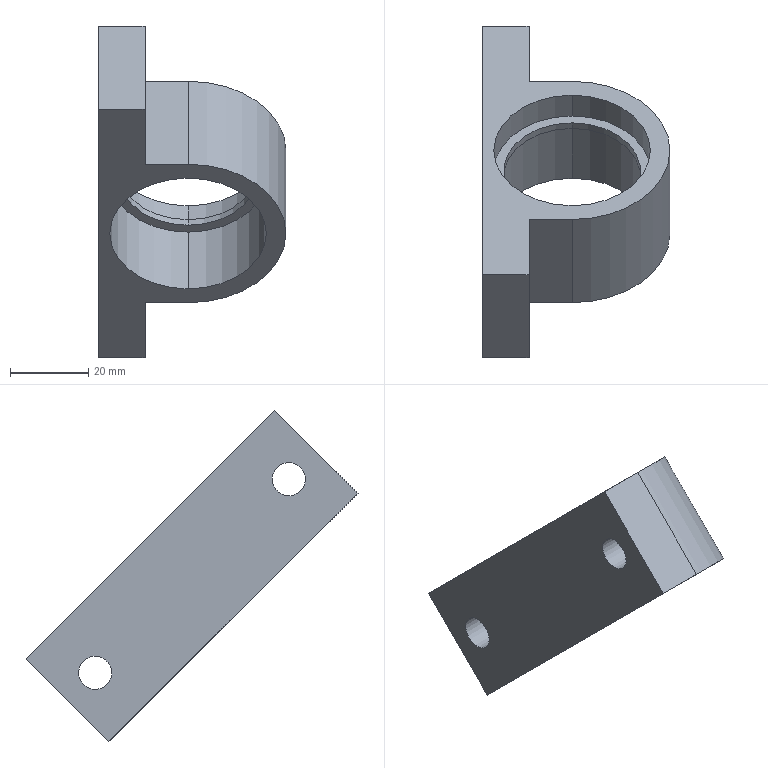Component | SolidWorks | AssemblyDriveAxis-1_BearingHousing6203-1 | 1 solid | 22 faces | box 48 x 84.85 x 84.85 mm | volume 39880 mm3 | cylinder 11 | plane 11 | commonest cylinder face diameters 40 x4 8.5 x4 35 x2 50 x1
build123d program:
from build123d import *

# Parameters (mm, degrees)
BOSS_EXTRUDE1_DEPTH            = 15
F_8_5_8_5_DIAMETER_HOLE1_D     = 8.5
F_8_5_8_5_DIAMETER_HOLE1_DEPTH = 52
F_8_5_8_5_DIAMETER_HOLE1_TIP   = 2.554
SKETCH6_R                      = 20
CUT_EXTRUDE1_DEPTH             = 7.5


with BuildPart() as part:
    # Sketch1 → Boss-Extrude1 (new, symmetric)
    with BuildSketch(Plane.XY):
        with BuildLine():
            Line((25, 17), (25, 6))
            Line((25, 6), (45, 6))
            Line((45, 6), (45, -6))
            Line((45, -6), (-45, -6))
            Line((-45, -6), (-45, 6))
            Line((-45, 6), (-25, 6))
            Line((-25, 6), (-25, 17))
            ThreePointArc((-25, 17), (0, 42), (25, 17))
        make_face()
    extrude(amount=BOSS_EXTRUDE1_DEPTH, both=True)

    # Sketch2 → Cut-Revolve1 (revolve, cut)
    with BuildSketch(Plane(origin=(0, 0, 0), x_dir=(0, 0, -1), z_dir=(1, 0, 0)), mode=Mode.PRIVATE) as cut_revolve1_sk:
        Polygon((15, 37), (8, 37), (6.5, 37), (-5.5, 37), (-5.5, 34.5), (-7.5, 34.5), (-7.5, 17), (15, 17), align=None)
    revolve(cut_revolve1_sk.sketch.rotate(Axis((0, 17, -34.227), (0, 0, 1)), 90), axis=Axis((0, 17, -34.227), (0, 0, 1)), mode=Mode.SUBTRACT)

    # 8.5 _8.5_ Diameter Hole1
    with Locations(Plane(origin=(0, 6, 0), x_dir=(1, 0, 0), z_dir=(0, 1, 0))):
        with Locations((35, 0), (-35, 0)):
            Hole(F_8_5_8_5_DIAMETER_HOLE1_D / 2, depth=F_8_5_8_5_DIAMETER_HOLE1_DEPTH)
            with Locations((0, 0, -(F_8_5_8_5_DIAMETER_HOLE1_DEPTH + F_8_5_8_5_DIAMETER_HOLE1_TIP / 2))):  # 118° drill point
                Cone(0, F_8_5_8_5_DIAMETER_HOLE1_D / 2, F_8_5_8_5_DIAMETER_HOLE1_TIP, mode=Mode.SUBTRACT)

    # Sketch6 → Cut-Extrude1 (cut)
    with BuildSketch(Plane.XY.offset(15)):
        with Locations(Location((0, 17, 0), (0, 0, 180))):
            Circle(SKETCH6_R)
    extrude(amount=-CUT_EXTRUDE1_DEPTH, mode=Mode.SUBTRACT)


solid = part.part

# Placed as in the assembly
solid = solid.moved(Location((-119, 778.165, 411.073), (-45, 0, -90)))
STEP:
#1=COLOUR_RGB('',0.7922,0.8196,0.9333);
#2=FILL_AREA_STYLE_COLOUR('',#1);
#3=FILL_AREA_STYLE('',(#2));
#4=SURFACE_STYLE_FILL_AREA(#3);
#5=SURFACE_SIDE_STYLE('',(#4));
#6=SURFACE_STYLE_USAGE(.BOTH.,#5);
#7=PRESENTATION_STYLE_ASSIGNMENT((#6));
#8=CARTESIAN_POINT('',(-4.016,31.402,15.836));
#9=VERTEX_POINT('',#8);
#10=CARTESIAN_POINT('',(-4.016,30.288,16.95));
#11=VERTEX_POINT('',#10);
#12=CARTESIAN_POINT('',(-4.016,30.845,16.393));
#13=DIRECTION('',(0.,0.7071,0.7071));
#14=DIRECTION('',(0.,-0.7071,0.7071));
#15=AXIS2_PLACEMENT_3D('',#12,#13,#14);
#16=CIRCLE('',#15,0.7874);
#17=EDGE_CURVE('',#9,#11,#16,.T.);
#18=ORIENTED_EDGE('',*,*,#17,.F.);
#19=CARTESIAN_POINT('',(-4.016,31.611,16.045));
#20=VERTEX_POINT('',#19);
#21=CARTESIAN_POINT('',(-4.016,31.402,15.836));
#22=DIRECTION('',(0.,0.7071,0.7071));
#23=VECTOR('',#22,39.37);
#24=LINE('',#21,#23);
#25=EDGE_CURVE('',#9,#20,#24,.T.);
#26=ORIENTED_EDGE('',*,*,#25,.T.);
#27=CARTESIAN_POINT('',(-4.016,30.497,17.158));
#28=VERTEX_POINT('',#27);
#29=CARTESIAN_POINT('',(-4.016,31.054,16.602));
#30=DIRECTION('',(0.,0.7071,0.7071));
#31=DIRECTION('',(0.,-0.7071,0.7071));
#32=AXIS2_PLACEMENT_3D('',#29,#30,#31);
#33=CIRCLE('',#32,0.7874);
#34=EDGE_CURVE('',#20,#28,#33,.T.);
#35=ORIENTED_EDGE('',*,*,#34,.T.);
#36=CARTESIAN_POINT('',(-4.016,30.288,16.95));
#37=DIRECTION('',(0.,0.7071,0.7071));
#38=VECTOR('',#37,39.37);
#39=LINE('',#36,#38);
#40=EDGE_CURVE('',#11,#28,#39,.T.);
#41=ORIENTED_EDGE('',*,*,#40,.F.);
#42=EDGE_LOOP('',(#18,#26,#35,#41));
#43=FACE_OUTER_BOUND('',#42,.T.);
#44=CARTESIAN_POINT('',(-4.016,30.845,16.393));
#45=DIRECTION('',(0.,0.7071,0.7071));
#46=DIRECTION('',(0.,-0.7071,0.7071));
#47=AXIS2_PLACEMENT_3D('',#44,#45,#46);
#48=CYLINDRICAL_SURFACE('',#47,0.7874);
#49=ADVANCED_FACE('',(#43),#48,.F.);
#50=CARTESIAN_POINT('',(-4.921,29.544,17.04));
#51=VERTEX_POINT('',#50);
#52=CARTESIAN_POINT('',(-4.921,29.78,17.277));
#53=VERTEX_POINT('',#52);
#54=CARTESIAN_POINT('',(-4.921,29.662,17.158));
#55=DIRECTION('',(1.,-0.,0.));
#56=DIRECTION('',(0.,0.7071,0.7071));
#57=AXIS2_PLACEMENT_3D('',#54,#55,#56);
#58=CIRCLE('',#57,0.1673);
#59=EDGE_CURVE('',#51,#53,#58,.T.);
#60=ORIENTED_EDGE('',*,*,#59,.F.);
#61=CARTESIAN_POINT('',(-4.449,29.544,17.04));
#62=VERTEX_POINT('',#61);
#63=CARTESIAN_POINT('',(-4.449,29.544,17.04));
#64=DIRECTION('',(1.,-0.,0.));
#65=VECTOR('',#64,39.37);
#66=LINE('',#63,#65);
#67=EDGE_CURVE('',#51,#62,#66,.T.);
#68=ORIENTED_EDGE('',*,*,#67,.T.);
#69=CARTESIAN_POINT('',(-4.449,29.78,17.277));
#70=VERTEX_POINT('',#69);
#71=CARTESIAN_POINT('',(-4.449,29.662,17.158));
#72=DIRECTION('',(1.,-0.,0.));
#73=DIRECTION('',(0.,0.7071,0.7071));
#74=AXIS2_PLACEMENT_3D('',#71,#72,#73);
#75=CIRCLE('',#74,0.1673);
#76=EDGE_CURVE('',#62,#70,#75,.T.);
#77=ORIENTED_EDGE('',*,*,#76,.T.);
#78=CARTESIAN_POINT('',(-4.449,29.78,17.277));
#79=DIRECTION('',(1.,-0.,0.));
#80=VECTOR('',#79,39.37);
#81=LINE('',#78,#80);
#82=EDGE_CURVE('',#53,#70,#81,.T.);
#83=ORIENTED_EDGE('',*,*,#82,.F.);
#84=EDGE_LOOP('',(#60,#68,#77,#83));
#85=FACE_OUTER_BOUND('',#84,.T.);
#86=CARTESIAN_POINT('',(-4.449,29.662,17.158));
#87=DIRECTION('',(1.,-0.,0.));
#88=DIRECTION('',(0.,0.7071,0.7071));
#89=AXIS2_PLACEMENT_3D('',#86,#87,#88);
#90=CYLINDRICAL_SURFACE('',#89,0.1673);
#91=ADVANCED_FACE('',(#85),#90,.F.);
#92=CARTESIAN_POINT('',(-4.921,31.492,15.091));
#93=VERTEX_POINT('',#92);
#94=CARTESIAN_POINT('',(-4.921,31.729,15.328));
#95=VERTEX_POINT('',#94);
#96=CARTESIAN_POINT('',(-4.921,31.611,15.21));
#97=DIRECTION('',(1.,-0.,0.));
#98=DIRECTION('',(0.,0.7071,0.7071));
#99=AXIS2_PLACEMENT_3D('',#96,#97,#98);
#100=CIRCLE('',#99,0.1673);
#101=EDGE_CURVE('',#93,#95,#100,.T.);
#102=ORIENTED_EDGE('',*,*,#101,.F.);
#103=CARTESIAN_POINT('',(-4.449,31.492,15.091));
#104=VERTEX_POINT('',#103);
#105=CARTESIAN_POINT('',(-4.449,31.492,15.091));
#106=DIRECTION('',(1.,-0.,0.));
#107=VECTOR('',#106,39.37);
#108=LINE('',#105,#107);
#109=EDGE_CURVE('',#93,#104,#108,.T.);
#110=ORIENTED_EDGE('',*,*,#109,.T.);
#111=CARTESIAN_POINT('',(-4.449,31.729,15.328));
#112=VERTEX_POINT('',#111);
#113=CARTESIAN_POINT('',(-4.449,31.611,15.21));
#114=DIRECTION('',(1.,-0.,0.));
#115=DIRECTION('',(0.,0.7071,0.7071));
#116=AXIS2_PLACEMENT_3D('',#113,#114,#115);
#117=CIRCLE('',#116,0.1673);
#118=EDGE_CURVE('',#104,#112,#117,.T.);
#119=ORIENTED_EDGE('',*,*,#118,.T.);
#120=CARTESIAN_POINT('',(-4.449,31.729,15.328));
#121=DIRECTION('',(1.,-0.,0.));
#122=VECTOR('',#121,39.37);
#123=LINE('',#120,#122);
#124=EDGE_CURVE('',#95,#112,#123,.T.);
#125=ORIENTED_EDGE('',*,*,#124,.F.);
#126=EDGE_LOOP('',(#102,#110,#119,#125));
#127=FACE_OUTER_BOUND('',#126,.T.);
#128=CARTESIAN_POINT('',(-4.449,31.611,15.21));
#129=DIRECTION('',(1.,-0.,0.));
#130=DIRECTION('',(0.,0.7071,0.7071));
#131=AXIS2_PLACEMENT_3D('',#128,#129,#130);
#132=CYLINDRICAL_SURFACE('',#131,0.1673);
#133=ADVANCED_FACE('',(#127),#132,.F.);
#134=CARTESIAN_POINT('',(-4.016,30.358,16.88));
#135=VERTEX_POINT('',#134);
#136=CARTESIAN_POINT('',(-4.016,31.332,15.906));
#137=VERTEX_POINT('',#136);
#138=CARTESIAN_POINT('',(-4.016,30.845,16.393));
#139=DIRECTION('',(0.,-0.7071,-0.7071));
#140=DIRECTION('',(0.,0.7071,-0.7071));
#141=AXIS2_PLACEMENT_3D('',#138,#139,#140);
#142=CIRCLE('',#141,0.689);
#143=EDGE_CURVE('',#135,#137,#142,.T.);
#144=ORIENTED_EDGE('',*,*,#143,.F.);
#145=CARTESIAN_POINT('',(-4.016,30.302,16.824));
#146=VERTEX_POINT('',#145);
#147=CARTESIAN_POINT('',(-4.016,29.196,15.718));
#148=DIRECTION('',(0.,-0.7071,-0.7071));
#149=VECTOR('',#148,39.37);
#150=LINE('',#147,#149);
#151=EDGE_CURVE('',#135,#146,#150,.T.);
#152=ORIENTED_EDGE('',*,*,#151,.T.);
#153=CARTESIAN_POINT('',(-4.016,31.277,15.85));
#154=VERTEX_POINT('',#153);
#155=CARTESIAN_POINT('',(-4.016,30.79,16.337));
#156=DIRECTION('',(0.,-0.7071,-0.7071));
#157=DIRECTION('',(0.,0.7071,-0.7071));
#158=AXIS2_PLACEMENT_3D('',#155,#156,#157);
#159=CIRCLE('',#158,0.689);
#160=EDGE_CURVE('',#146,#154,#159,.T.);
#161=ORIENTED_EDGE('',*,*,#160,.T.);
#162=CARTESIAN_POINT('',(-4.016,30.171,14.744));
#163=DIRECTION('',(0.,-0.7071,-0.7071));
#164=VECTOR('',#163,39.37);
#165=LINE('',#162,#164);
#166=EDGE_CURVE('',#137,#154,#165,.T.);
#167=ORIENTED_EDGE('',*,*,#166,.F.);
#168=EDGE_LOOP('',(#144,#152,#161,#167));
#169=FACE_OUTER_BOUND('',#168,.T.);
#170=CARTESIAN_POINT('',(-4.016,29.684,15.231));
#171=DIRECTION('',(0.,-0.7071,-0.7071));
#172=DIRECTION('',(0.,0.7071,-0.7071));
#173=AXIS2_PLACEMENT_3D('',#170,#171,#172);
#174=CYLINDRICAL_SURFACE('',#173,0.689);
#175=ADVANCED_FACE('',(#169),#174,.F.);
#176=CARTESIAN_POINT('',(-4.016,30.233,16.894));
#177=VERTEX_POINT('',#176);
#178=CARTESIAN_POINT('',(-4.016,31.346,15.78));
#179=VERTEX_POINT('',#178);
#180=CARTESIAN_POINT('',(-4.016,30.79,16.337));
#181=DIRECTION('',(0.,-0.7071,-0.7071));
#182=DIRECTION('',(0.,0.7071,-0.7071));
#183=AXIS2_PLACEMENT_3D('',#180,#181,#182);
#184=CIRCLE('',#183,0.7874);
#185=EDGE_CURVE('',#177,#179,#184,.T.);
#186=ORIENTED_EDGE('',*,*,#185,.F.);
#187=CARTESIAN_POINT('',(-4.016,29.662,16.323));
#188=VERTEX_POINT('',#187);
#189=CARTESIAN_POINT('',(-4.016,29.127,15.788));
#190=DIRECTION('',(0.,-0.7071,-0.7071));
#191=VECTOR('',#190,39.37);
#192=LINE('',#189,#191);
#193=EDGE_CURVE('',#177,#188,#192,.T.);
#194=ORIENTED_EDGE('',*,*,#193,.T.);
#195=CARTESIAN_POINT('',(-4.016,30.776,15.21));
#196=VERTEX_POINT('',#195);
#197=CARTESIAN_POINT('',(-4.016,30.219,15.766));
#198=DIRECTION('',(0.,-0.7071,-0.7071));
#199=DIRECTION('',(0.,0.7071,-0.7071));
#200=AXIS2_PLACEMENT_3D('',#197,#198,#199);
#201=CIRCLE('',#200,0.7874);
#202=EDGE_CURVE('',#188,#196,#201,.T.);
#203=ORIENTED_EDGE('',*,*,#202,.T.);
#204=CARTESIAN_POINT('',(-4.016,30.24,14.674));
#205=DIRECTION('',(0.,-0.7071,-0.7071));
#206=VECTOR('',#205,39.37);
#207=LINE('',#204,#206);
#208=EDGE_CURVE('',#179,#196,#207,.T.);
#209=ORIENTED_EDGE('',*,*,#208,.F.);
#210=EDGE_LOOP('',(#186,#194,#203,#209));
#211=FACE_OUTER_BOUND('',#210,.T.);
#212=CARTESIAN_POINT('',(-4.016,29.684,15.231));
#213=DIRECTION('',(0.,-0.7071,-0.7071));
#214=DIRECTION('',(0.,0.7071,-0.7071));
#215=AXIS2_PLACEMENT_3D('',#212,#213,#214);
#216=CYLINDRICAL_SURFACE('',#215,0.7874);
#217=ADVANCED_FACE('',(#211),#216,.F.);
#218=CARTESIAN_POINT('',(-4.921,28.966,17.019));
#219=VERTEX_POINT('',#218);
#220=CARTESIAN_POINT('',(-4.449,28.966,17.019));
#221=VERTEX_POINT('',#220);
#222=CARTESIAN_POINT('',(-4.449,28.966,17.019));
#223=DIRECTION('',(1.,-0.,0.));
#224=VECTOR('',#223,39.37);
#225=LINE('',#222,#224);
#226=EDGE_CURVE('',#219,#221,#225,.T.);
#227=ORIENTED_EDGE('',*,*,#226,.T.);
#228=CARTESIAN_POINT('',(-4.449,29.801,17.854));
#229=VERTEX_POINT('',#228);
#230=CARTESIAN_POINT('',(-4.449,29.801,17.854));
#231=DIRECTION('',(0.,-0.7071,-0.7071));
#232=VECTOR('',#231,39.37);
#233=LINE('',#230,#232);
#234=EDGE_CURVE('',#229,#221,#233,.T.);
#235=ORIENTED_EDGE('',*,*,#234,.F.);
#236=CARTESIAN_POINT('',(-4.921,29.801,17.854));
#237=VERTEX_POINT('',#236);
#238=CARTESIAN_POINT('',(-4.449,29.801,17.854));
#239=DIRECTION('',(1.,-0.,0.));
#240=VECTOR('',#239,39.37);
#241=LINE('',#238,#240);
#242=EDGE_CURVE('',#237,#229,#241,.T.);
#243=ORIENTED_EDGE('',*,*,#242,.F.);
#244=CARTESIAN_POINT('',(-4.921,29.801,17.854));
#245=DIRECTION('',(0.,-0.7071,-0.7071));
#246=VECTOR('',#245,39.37);
#247=LINE('',#244,#246);
#248=EDGE_CURVE('',#237,#219,#247,.T.);
#249=ORIENTED_EDGE('',*,*,#248,.T.);
#250=EDGE_LOOP('',(#227,#235,#243,#249));
#251=FACE_OUTER_BOUND('',#250,.T.);
#252=CARTESIAN_POINT('',(-4.449,29.801,17.854));
#253=DIRECTION('',(0.,0.7071,-0.7071));
#254=DIRECTION('',(0.,0.7071,0.7071));
#255=AXIS2_PLACEMENT_3D('',#252,#253,#254);
#256=PLANE('',#255);
#257=ADVANCED_FACE('',(#251),#256,.F.);
#258=CARTESIAN_POINT('',(-4.449,29.662,17.158));
#259=DIRECTION('',(1.,-0.,0.));
#260=DIRECTION('',(0.,0.7071,0.7071));
#261=AXIS2_PLACEMENT_3D('',#258,#259,#260);
#262=CIRCLE('',#261,0.1673);
#263=EDGE_CURVE('',#70,#62,#262,.T.);
#264=ORIENTED_EDGE('',*,*,#263,.F.);
#265=ORIENTED_EDGE('',*,*,#76,.F.);
#266=EDGE_LOOP('',(#264,#265));
#267=FACE_BOUND('',#266,.T.);
#268=CARTESIAN_POINT('',(-4.449,29.523,16.462));
#269=VERTEX_POINT('',#268);
#270=CARTESIAN_POINT('',(-4.449,29.523,16.462));
#271=DIRECTION('',(0.,0.7071,-0.7071));
#272=VECTOR('',#271,39.37);
#273=LINE('',#270,#272);
#274=EDGE_CURVE('',#221,#269,#273,.T.);
#275=ORIENTED_EDGE('',*,*,#274,.T.);
#276=CARTESIAN_POINT('',(-4.449,30.358,17.298));
#277=VERTEX_POINT('',#276);
#278=CARTESIAN_POINT('',(-4.449,30.358,17.298));
#279=DIRECTION('',(0.,-0.7071,-0.7071));
#280=VECTOR('',#279,39.37);
#281=LINE('',#278,#280);
#282=EDGE_CURVE('',#277,#269,#281,.T.);
#283=ORIENTED_EDGE('',*,*,#282,.F.);
#284=CARTESIAN_POINT('',(-4.449,30.358,17.298));
#285=DIRECTION('',(0.,0.7071,-0.7071));
#286=VECTOR('',#285,39.37);
#287=LINE('',#284,#286);
#288=EDGE_CURVE('',#229,#277,#287,.T.);
#289=ORIENTED_EDGE('',*,*,#288,.F.);
#290=ORIENTED_EDGE('',*,*,#234,.T.);
#291=EDGE_LOOP('',(#275,#283,#289,#290));
#292=FACE_OUTER_BOUND('',#291,.T.);
#293=CARTESIAN_POINT('',(-4.449,30.358,17.298));
#294=DIRECTION('',(-1.,0.,-0.));
#295=DIRECTION('',(-0.,-0.7071,0.7071));
#296=AXIS2_PLACEMENT_3D('',#293,#294,#295);
#297=PLANE('',#296);
#298=ADVANCED_FACE('',(#267,#292),#297,.F.);
#299=CARTESIAN_POINT('',(-4.016,29.523,16.462));
#300=VERTEX_POINT('',#299);
#301=CARTESIAN_POINT('',(-4.016,29.523,16.462));
#302=DIRECTION('',(1.,-0.,0.));
#303=VECTOR('',#302,39.37);
#304=LINE('',#301,#303);
#305=EDGE_CURVE('',#269,#300,#304,.T.);
#306=ORIENTED_EDGE('',*,*,#305,.T.);
#307=CARTESIAN_POINT('',(-4.016,30.358,17.298));
#308=VERTEX_POINT('',#307);
#309=CARTESIAN_POINT('',(-4.016,30.358,17.298));
#310=DIRECTION('',(0.,-0.7071,-0.7071));
#311=VECTOR('',#310,39.37);
#312=LINE('',#309,#311);
#313=EDGE_CURVE('',#308,#300,#312,.T.);
#314=ORIENTED_EDGE('',*,*,#313,.F.);
#315=CARTESIAN_POINT('',(-4.016,30.358,17.298));
#316=DIRECTION('',(1.,-0.,0.));
#317=VECTOR('',#316,39.37);
#318=LINE('',#315,#317);
#319=EDGE_CURVE('',#277,#308,#318,.T.);
#320=ORIENTED_EDGE('',*,*,#319,.F.);
#321=ORIENTED_EDGE('',*,*,#282,.T.);
#322=EDGE_LOOP('',(#306,#314,#320,#321));
#323=FACE_OUTER_BOUND('',#322,.T.);
#324=CARTESIAN_POINT('',(-4.016,30.358,17.298));
#325=DIRECTION('',(0.,0.7071,-0.7071));
#326=DIRECTION('',(-1.,0.,-0.));
#327=AXIS2_PLACEMENT_3D('',#324,#325,#326);
#328=PLANE('',#327);
#329=ADVANCED_FACE('',(#323),#328,.F.);
#330=CARTESIAN_POINT('',(-4.016,30.915,15.07));
#331=VERTEX_POINT('',#330);
#332=CARTESIAN_POINT('',(-4.016,30.219,15.766));
#333=DIRECTION('',(0.,0.7071,0.7071));
#334=DIRECTION('',(0.,-0.7071,0.7071));
#335=AXIS2_PLACEMENT_3D('',#332,#333,#334);
#336=CIRCLE('',#335,0.9843);
#337=EDGE_CURVE('',#300,#331,#336,.T.);
#338=ORIENTED_EDGE('',*,*,#337,.T.);
#339=CARTESIAN_POINT('',(-4.016,31.75,15.906));
#340=VERTEX_POINT('',#339);
#341=CARTESIAN_POINT('',(-4.016,31.75,15.906));
#342=DIRECTION('',(0.,-0.7071,-0.7071));
#343=VECTOR('',#342,39.37);
#344=LINE('',#341,#343);
#345=EDGE_CURVE('',#340,#331,#344,.T.);
#346=ORIENTED_EDGE('',*,*,#345,.F.);
#347=CARTESIAN_POINT('',(-4.016,31.054,16.602));
#348=DIRECTION('',(0.,0.7071,0.7071));
#349=DIRECTION('',(0.,-0.7071,0.7071));
#350=AXIS2_PLACEMENT_3D('',#347,#348,#349);
#351=CIRCLE('',#350,0.9843);
#352=EDGE_CURVE('',#308,#340,#351,.T.);
#353=ORIENTED_EDGE('',*,*,#352,.F.);
#354=ORIENTED_EDGE('',*,*,#313,.T.);
#355=EDGE_LOOP('',(#338,#346,#353,#354));
#356=FACE_OUTER_BOUND('',#355,.T.);
#357=CARTESIAN_POINT('',(-4.016,31.054,16.602));
#358=DIRECTION('',(0.,-0.7071,-0.7071));
#359=DIRECTION('',(0.,0.7071,-0.7071));
#360=AXIS2_PLACEMENT_3D('',#357,#358,#359);
#361=CYLINDRICAL_SURFACE('',#360,0.9843);
#362=ADVANCED_FACE('',(#356),#361,.T.);
#363=CARTESIAN_POINT('',(-4.449,30.915,15.07));
#364=VERTEX_POINT('',#363);
#365=CARTESIAN_POINT('',(-4.016,30.915,15.07));
#366=DIRECTION('',(-1.,-0.,0.));
#367=VECTOR('',#366,39.37);
#368=LINE('',#365,#367);
#369=EDGE_CURVE('',#331,#364,#368,.T.);
#370=ORIENTED_EDGE('',*,*,#369,.T.);
#371=CARTESIAN_POINT('',(-4.449,31.75,15.906));
#372=VERTEX_POINT('',#371);
#373=CARTESIAN_POINT('',(-4.449,31.75,15.906));
#374=DIRECTION('',(0.,-0.7071,-0.7071));
#375=VECTOR('',#374,39.37);
#376=LINE('',#373,#375);
#377=EDGE_CURVE('',#372,#364,#376,.T.);
#378=ORIENTED_EDGE('',*,*,#377,.F.);
#379=CARTESIAN_POINT('',(-4.016,31.75,15.906));
#380=DIRECTION('',(-1.,-0.,0.));
#381=VECTOR('',#380,39.37);
#382=LINE('',#379,#381);
#383=EDGE_CURVE('',#340,#372,#382,.T.);
#384=ORIENTED_EDGE('',*,*,#383,.F.);
#385=ORIENTED_EDGE('',*,*,#345,.T.);
#386=EDGE_LOOP('',(#370,#378,#384,#385));
#387=FACE_OUTER_BOUND('',#386,.T.);
#388=CARTESIAN_POINT('',(-4.016,31.75,15.906));
#389=DIRECTION('',(0.,-0.7071,0.7071));
#390=DIRECTION('',(1.,0.,-0.));
#391=AXIS2_PLACEMENT_3D('',#388,#389,#390);
#392=PLANE('',#391);
#393=ADVANCED_FACE('',(#387),#392,.F.);
#394=CARTESIAN_POINT('',(-4.449,31.611,15.21));
#395=DIRECTION('',(1.,-0.,0.));
#396=DIRECTION('',(0.,0.7071,0.7071));
#397=AXIS2_PLACEMENT_3D('',#394,#395,#396);
#398=CIRCLE('',#397,0.1673);
#399=EDGE_CURVE('',#112,#104,#398,.T.);
#400=ORIENTED_EDGE('',*,*,#399,.F.);
#401=ORIENTED_EDGE('',*,*,#118,.F.);
#402=EDGE_LOOP('',(#400,#401));
#403=FACE_BOUND('',#402,.T.);
#404=CARTESIAN_POINT('',(-4.449,31.472,14.514));
#405=VERTEX_POINT('',#404);
#406=CARTESIAN_POINT('',(-4.449,31.472,14.514));
#407=DIRECTION('',(0.,0.7071,-0.7071));
#408=VECTOR('',#407,39.37);
#409=LINE('',#406,#408);
#410=EDGE_CURVE('',#364,#405,#409,.T.);
#411=ORIENTED_EDGE('',*,*,#410,.T.);
#412=CARTESIAN_POINT('',(-4.449,32.307,15.349));
#413=VERTEX_POINT('',#412);
#414=CARTESIAN_POINT('',(-4.449,32.307,15.349));
#415=DIRECTION('',(0.,-0.7071,-0.7071));
#416=VECTOR('',#415,39.37);
#417=LINE('',#414,#416);
#418=EDGE_CURVE('',#413,#405,#417,.T.);
#419=ORIENTED_EDGE('',*,*,#418,.F.);
#420=CARTESIAN_POINT('',(-4.449,32.307,15.349));
#421=DIRECTION('',(0.,0.7071,-0.7071));
#422=VECTOR('',#421,39.37);
#423=LINE('',#420,#422);
#424=EDGE_CURVE('',#372,#413,#423,.T.);
#425=ORIENTED_EDGE('',*,*,#424,.F.);
#426=ORIENTED_EDGE('',*,*,#377,.T.);
#427=EDGE_LOOP('',(#411,#419,#425,#426));
#428=FACE_OUTER_BOUND('',#427,.T.);
#429=CARTESIAN_POINT('',(-4.449,32.307,15.349));
#430=DIRECTION('',(-1.,0.,-0.));
#431=DIRECTION('',(0.,-0.7071,-0.7071));
#432=AXIS2_PLACEMENT_3D('',#429,#430,#431);
#433=PLANE('',#432);
#434=ADVANCED_FACE('',(#403,#428),#433,.F.);
#435=CARTESIAN_POINT('',(-4.921,31.472,14.514));
#436=VERTEX_POINT('',#435);
#437=CARTESIAN_POINT('',(-4.449,31.472,14.514));
#438=DIRECTION('',(-1.,0.,-0.));
#439=VECTOR('',#438,39.37);
#440=LINE('',#437,#439);
#441=EDGE_CURVE('',#405,#436,#440,.T.);
#442=ORIENTED_EDGE('',*,*,#441,.T.);
#443=CARTESIAN_POINT('',(-4.921,32.307,15.349));
#444=VERTEX_POINT('',#443);
#445=CARTESIAN_POINT('',(-4.921,32.307,15.349));
#446=DIRECTION('',(0.,-0.7071,-0.7071));
#447=VECTOR('',#446,39.37);
#448=LINE('',#445,#447);
#449=EDGE_CURVE('',#444,#436,#448,.T.);
#450=ORIENTED_EDGE('',*,*,#449,.F.);
#451=CARTESIAN_POINT('',(-4.449,32.307,15.349));
#452=DIRECTION('',(-1.,0.,-0.));
#453=VECTOR('',#452,39.37);
#454=LINE('',#451,#453);
#455=EDGE_CURVE('',#413,#444,#454,.T.);
#456=ORIENTED_EDGE('',*,*,#455,.F.);
#457=ORIENTED_EDGE('',*,*,#418,.T.);
#458=EDGE_LOOP('',(#442,#450,#456,#457));
#459=FACE_OUTER_BOUND('',#458,.T.);
#460=CARTESIAN_POINT('',(-4.449,32.307,15.349));
#461=DIRECTION('',(-0.,-0.7071,0.7071));
#462=DIRECTION('',(0.,-0.7071,-0.7071));
#463=AXIS2_PLACEMENT_3D('',#460,#461,#462);
#464=PLANE('',#463);
#465=ADVANCED_FACE('',(#459),#464,.F.);
#466=CARTESIAN_POINT('',(-4.921,29.662,17.158));
#467=DIRECTION('',(1.,-0.,0.));
#468=DIRECTION('',(0.,0.7071,0.7071));
#469=AXIS2_PLACEMENT_3D('',#466,#467,#468);
#470=CIRCLE('',#469,0.1673);
#471=EDGE_CURVE('',#53,#51,#470,.T.);
#472=ORIENTED_EDGE('',*,*,#471,.T.);
#473=ORIENTED_EDGE('',*,*,#59,.T.);
#474=EDGE_LOOP('',(#472,#473));
#475=FACE_BOUND('',#474,.T.);
#476=CARTESIAN_POINT('',(-4.921,31.611,15.21));
#477=DIRECTION('',(1.,-0.,0.));
#478=DIRECTION('',(0.,0.7071,0.7071));
#479=AXIS2_PLACEMENT_3D('',#476,#477,#478);
#480=CIRCLE('',#479,0.1673);
#481=EDGE_CURVE('',#95,#93,#480,.T.);
#482=ORIENTED_EDGE('',*,*,#481,.T.);
#483=ORIENTED_EDGE('',*,*,#101,.T.);
#484=EDGE_LOOP('',(#482,#483));
#485=FACE_BOUND('',#484,.T.);
#486=CARTESIAN_POINT('',(-4.921,31.472,14.514));
#487=DIRECTION('',(-0.,-0.7071,0.7071));
#488=VECTOR('',#487,39.37);
#489=LINE('',#486,#488);
#490=EDGE_CURVE('',#436,#219,#489,.T.);
#491=ORIENTED_EDGE('',*,*,#490,.T.);
#492=ORIENTED_EDGE('',*,*,#248,.F.);
#493=CARTESIAN_POINT('',(-4.921,32.307,15.349));
#494=DIRECTION('',(-0.,-0.7071,0.7071));
#495=VECTOR('',#494,39.37);
#496=LINE('',#493,#495);
#497=EDGE_CURVE('',#444,#237,#496,.T.);
#498=ORIENTED_EDGE('',*,*,#497,.F.);
#499=ORIENTED_EDGE('',*,*,#449,.T.);
#500=EDGE_LOOP('',(#491,#492,#498,#499));
#501=FACE_OUTER_BOUND('',#500,.T.);
#502=CARTESIAN_POINT('',(-4.921,32.307,15.349));
#503=DIRECTION('',(1.,-0.,0.));
#504=DIRECTION('',(0.,0.7071,0.7071));
#505=AXIS2_PLACEMENT_3D('',#502,#503,#504);
#506=PLANE('',#505);
#507=ADVANCED_FACE('',(#475,#485,#501),#506,.F.);
#508=CARTESIAN_POINT('',(-4.016,31.054,16.602));
#509=DIRECTION('',(0.,0.7071,0.7071));
#510=DIRECTION('',(0.,-0.7071,0.7071));
#511=AXIS2_PLACEMENT_3D('',#508,#509,#510);
#512=CIRCLE('',#511,0.7874);
#513=EDGE_CURVE('',#28,#20,#512,.T.);
#514=ORIENTED_EDGE('',*,*,#513,.F.);
#515=ORIENTED_EDGE('',*,*,#34,.F.);
#516=EDGE_LOOP('',(#514,#515));
#517=FACE_BOUND('',#516,.T.);
#518=ORIENTED_EDGE('',*,*,#242,.T.);
#519=ORIENTED_EDGE('',*,*,#288,.T.);
#520=ORIENTED_EDGE('',*,*,#319,.T.);
#521=ORIENTED_EDGE('',*,*,#352,.T.);
#522=ORIENTED_EDGE('',*,*,#383,.T.);
#523=ORIENTED_EDGE('',*,*,#424,.T.);
#524=ORIENTED_EDGE('',*,*,#455,.T.);
#525=ORIENTED_EDGE('',*,*,#497,.T.);
#526=EDGE_LOOP('',(#518,#519,#520,#521,#522,#523,#524,#525));
#527=FACE_OUTER_BOUND('',#526,.T.);
#528=CARTESIAN_POINT('',(-4.016,31.054,16.602));
#529=DIRECTION('',(0.,0.7071,0.7071));
#530=DIRECTION('',(-0.,-0.7071,0.7071));
#531=AXIS2_PLACEMENT_3D('',#528,#529,#530);
#532=PLANE('',#531);
#533=ADVANCED_FACE('',(#517,#527),#532,.T.);
#534=CARTESIAN_POINT('',(-4.016,30.219,15.766));
#535=DIRECTION('',(0.,-0.7071,-0.7071));
#536=DIRECTION('',(0.,0.7071,-0.7071));
#537=AXIS2_PLACEMENT_3D('',#534,#535,#536);
#538=CIRCLE('',#537,0.7874);
#539=EDGE_CURVE('',#196,#188,#538,.T.);
#540=ORIENTED_EDGE('',*,*,#539,.F.);
#541=ORIENTED_EDGE('',*,*,#202,.F.);
#542=EDGE_LOOP('',(#540,#541));
#543=FACE_BOUND('',#542,.T.);
#544=ORIENTED_EDGE('',*,*,#226,.F.);
#545=ORIENTED_EDGE('',*,*,#490,.F.);
#546=ORIENTED_EDGE('',*,*,#441,.F.);
#547=ORIENTED_EDGE('',*,*,#410,.F.);
#548=ORIENTED_EDGE('',*,*,#369,.F.);
#549=ORIENTED_EDGE('',*,*,#337,.F.);
#550=ORIENTED_EDGE('',*,*,#305,.F.);
#551=ORIENTED_EDGE('',*,*,#274,.F.);
#552=EDGE_LOOP('',(#544,#545,#546,#547,#548,#549,#550,#551));
#553=FACE_OUTER_BOUND('',#552,.T.);
#554=CARTESIAN_POINT('',(-4.016,30.219,15.766));
#555=DIRECTION('',(0.,0.7071,0.7071));
#556=DIRECTION('',(-0.,-0.7071,0.7071));
#557=AXIS2_PLACEMENT_3D('',#554,#555,#556);
#558=PLANE('',#557);
#559=ADVANCED_FACE('',(#543,#553),#558,.F.);
#560=ORIENTED_EDGE('',*,*,#193,.F.);
#561=CARTESIAN_POINT('',(-4.016,30.79,16.337));
#562=DIRECTION('',(0.,-0.7071,-0.7071));
#563=DIRECTION('',(0.,0.7071,-0.7071));
#564=AXIS2_PLACEMENT_3D('',#561,#562,#563);
#565=CIRCLE('',#564,0.7874);
#566=EDGE_CURVE('',#179,#177,#565,.T.);
#567=ORIENTED_EDGE('',*,*,#566,.F.);
#568=ORIENTED_EDGE('',*,*,#208,.T.);
#569=ORIENTED_EDGE('',*,*,#539,.T.);
#570=EDGE_LOOP('',(#560,#567,#568,#569));
#571=FACE_OUTER_BOUND('',#570,.T.);
#572=CARTESIAN_POINT('',(-4.016,29.684,15.231));
#573=DIRECTION('',(0.,-0.7071,-0.7071));
#574=DIRECTION('',(0.,0.7071,-0.7071));
#575=AXIS2_PLACEMENT_3D('',#572,#573,#574);
#576=CYLINDRICAL_SURFACE('',#575,0.7874);
#577=ADVANCED_FACE('',(#571),#576,.F.);
#578=CARTESIAN_POINT('',(-4.016,30.79,16.337));
#579=DIRECTION('',(0.,-0.7071,-0.7071));
#580=DIRECTION('',(0.,0.7071,-0.7071));
#581=AXIS2_PLACEMENT_3D('',#578,#579,#580);
#582=CIRCLE('',#581,0.689);
#583=EDGE_CURVE('',#154,#146,#582,.T.);
#584=ORIENTED_EDGE('',*,*,#583,.F.);
#585=ORIENTED_EDGE('',*,*,#160,.F.);
#586=EDGE_LOOP('',(#584,#585));
#587=FACE_BOUND('',#586,.T.);
#588=ORIENTED_EDGE('',*,*,#566,.T.);
#589=ORIENTED_EDGE('',*,*,#185,.T.);
#590=EDGE_LOOP('',(#588,#589));
#591=FACE_OUTER_BOUND('',#590,.T.);
#592=CARTESIAN_POINT('',(-3.228,30.79,16.337));
#593=DIRECTION('',(0.,0.7071,0.7071));
#594=DIRECTION('',(-0.,-0.7071,0.7071));
#595=AXIS2_PLACEMENT_3D('',#592,#593,#594);
#596=PLANE('',#595);
#597=ADVANCED_FACE('',(#587,#591),#596,.F.);
#598=ORIENTED_EDGE('',*,*,#151,.F.);
#599=CARTESIAN_POINT('',(-4.016,30.845,16.393));
#600=DIRECTION('',(0.,-0.7071,-0.7071));
#601=DIRECTION('',(0.,0.7071,-0.7071));
#602=AXIS2_PLACEMENT_3D('',#599,#600,#601);
#603=CIRCLE('',#602,0.689);
#604=EDGE_CURVE('',#137,#135,#603,.T.);
#605=ORIENTED_EDGE('',*,*,#604,.F.);
#606=ORIENTED_EDGE('',*,*,#166,.T.);
#607=ORIENTED_EDGE('',*,*,#583,.T.);
#608=EDGE_LOOP('',(#598,#605,#606,#607));
#609=FACE_OUTER_BOUND('',#608,.T.);
#610=CARTESIAN_POINT('',(-4.016,29.684,15.231));
#611=DIRECTION('',(0.,-0.7071,-0.7071));
#612=DIRECTION('',(0.,0.7071,-0.7071));
#613=AXIS2_PLACEMENT_3D('',#610,#611,#612);
#614=CYLINDRICAL_SURFACE('',#613,0.689);
#615=ADVANCED_FACE('',(#609),#614,.F.);
#616=ORIENTED_EDGE('',*,*,#109,.F.);
#617=ORIENTED_EDGE('',*,*,#481,.F.);
#618=ORIENTED_EDGE('',*,*,#124,.T.);
#619=ORIENTED_EDGE('',*,*,#399,.T.);
#620=EDGE_LOOP('',(#616,#617,#618,#619));
#621=FACE_OUTER_BOUND('',#620,.T.);
#622=CARTESIAN_POINT('',(-4.449,31.611,15.21));
#623=DIRECTION('',(1.,-0.,0.));
#624=DIRECTION('',(0.,0.7071,0.7071));
#625=AXIS2_PLACEMENT_3D('',#622,#623,#624);
#626=CYLINDRICAL_SURFACE('',#625,0.1673);
#627=ADVANCED_FACE('',(#621),#626,.F.);
#628=ORIENTED_EDGE('',*,*,#67,.F.);
#629=ORIENTED_EDGE('',*,*,#471,.F.);
#630=ORIENTED_EDGE('',*,*,#82,.T.);
#631=ORIENTED_EDGE('',*,*,#263,.T.);
#632=EDGE_LOOP('',(#628,#629,#630,#631));
#633=FACE_OUTER_BOUND('',#632,.T.);
#634=CARTESIAN_POINT('',(-4.449,29.662,17.158));
#635=DIRECTION('',(1.,-0.,0.));
#636=DIRECTION('',(0.,0.7071,0.7071));
#637=AXIS2_PLACEMENT_3D('',#634,#635,#636);
#638=CYLINDRICAL_SURFACE('',#637,0.1673);
#639=ADVANCED_FACE('',(#633),#638,.F.);
#640=CARTESIAN_POINT('',(-4.016,30.845,16.393));
#641=DIRECTION('',(0.,0.7071,0.7071));
#642=DIRECTION('',(0.,-0.7071,0.7071));
#643=AXIS2_PLACEMENT_3D('',#640,#641,#642);
#644=CIRCLE('',#643,0.7874);
#645=EDGE_CURVE('',#11,#9,#644,.T.);
#646=ORIENTED_EDGE('',*,*,#645,.T.);
#647=ORIENTED_EDGE('',*,*,#17,.T.);
#648=EDGE_LOOP('',(#646,#647));
#649=FACE_OUTER_BOUND('',#648,.T.);
#650=ORIENTED_EDGE('',*,*,#604,.T.);
#651=ORIENTED_EDGE('',*,*,#143,.T.);
#652=EDGE_LOOP('',(#650,#651));
#653=FACE_BOUND('',#652,.T.);
#654=CARTESIAN_POINT('',(-4.016,30.845,16.393));
#655=DIRECTION('',(0.,0.7071,0.7071));
#656=DIRECTION('',(-0.,-0.7071,0.7071));
#657=AXIS2_PLACEMENT_3D('',#654,#655,#656);
#658=PLANE('',#657);
#659=ADVANCED_FACE('',(#649,#653),#658,.T.);
#660=ORIENTED_EDGE('',*,*,#25,.F.);
#661=ORIENTED_EDGE('',*,*,#645,.F.);
#662=ORIENTED_EDGE('',*,*,#40,.T.);
#663=ORIENTED_EDGE('',*,*,#513,.T.);
#664=EDGE_LOOP('',(#660,#661,#662,#663));
#665=FACE_OUTER_BOUND('',#664,.T.);
#666=CARTESIAN_POINT('',(-4.016,30.845,16.393));
#667=DIRECTION('',(0.,0.7071,0.7071));
#668=DIRECTION('',(0.,-0.7071,0.7071));
#669=AXIS2_PLACEMENT_3D('',#666,#667,#668);
#670=CYLINDRICAL_SURFACE('',#669,0.7874);
#671=ADVANCED_FACE('',(#665),#670,.F.);
#672=CLOSED_SHELL('',(#49,#91,#133,#175,#217,#257,#298,#329,#362,#393,#434,#465,#507,#533,#559,#577,#597,#615,#627,#639,#659,#671));
#673=MANIFOLD_SOLID_BREP('',#672);
#674=STYLED_ITEM('',(#7),#673);
#675=(LENGTH_UNIT()NAMED_UNIT(*)SI_UNIT($,.METRE.));
#676=LENGTH_MEASURE_WITH_UNIT(LENGTH_MEASURE(0.0254),#675);
#677=DIMENSIONAL_EXPONENTS(1.,0.,0.,0.,0.,0.,0.);
#678=(CONVERSION_BASED_UNIT('',#676)LENGTH_UNIT()NAMED_UNIT(#677));
#679=UNCERTAINTY_MEASURE_WITH_UNIT(LENGTH_MEASURE(0.00001),#678,'','');
#680=(NAMED_UNIT(*)PLANE_ANGLE_UNIT()SI_UNIT($,.RADIAN.));
#681=(NAMED_UNIT(*)SI_UNIT($,.STERADIAN.)SOLID_ANGLE_UNIT());
#682=(GEOMETRIC_REPRESENTATION_CONTEXT(3)GLOBAL_UNCERTAINTY_ASSIGNED_CONTEXT((#679))GLOBAL_UNIT_ASSIGNED_CONTEXT((#678,#680,#681))REPRESENTATION_CONTEXT('',''));
#683=MECHANICAL_DESIGN_GEOMETRIC_PRESENTATION_REPRESENTATION('',(#674),#682);
#684=CARTESIAN_POINT('',(0.,0.,0.));
#685=DIRECTION('',(0.,0.,1.));
#686=DIRECTION('',(1.,0.,0.));
#687=AXIS2_PLACEMENT_3D('',#684,#685,#686);
#688=(LENGTH_UNIT()NAMED_UNIT(*)SI_UNIT($,.METRE.));
#689=LENGTH_MEASURE_WITH_UNIT(LENGTH_MEASURE(0.0254),#688);
#690=DIMENSIONAL_EXPONENTS(1.,0.,0.,0.,0.,0.,0.);
#691=(CONVERSION_BASED_UNIT('',#689)LENGTH_UNIT()NAMED_UNIT(#690));
#692=UNCERTAINTY_MEASURE_WITH_UNIT(LENGTH_MEASURE(0.00001),#691,'','');
#693=(NAMED_UNIT(*)PLANE_ANGLE_UNIT()SI_UNIT($,.RADIAN.));
#694=(NAMED_UNIT(*)SI_UNIT($,.STERADIAN.)SOLID_ANGLE_UNIT());
#695=(GEOMETRIC_REPRESENTATION_CONTEXT(3)GLOBAL_UNCERTAINTY_ASSIGNED_CONTEXT((#692))GLOBAL_UNIT_ASSIGNED_CONTEXT((#691,#693,#694))REPRESENTATION_CONTEXT('',''));
#696=ADVANCED_BREP_SHAPE_REPRESENTATION('',(#673,#687),#695);
#697=PRESENTATION_LAYER_ASSIGNMENT('','',(#674));